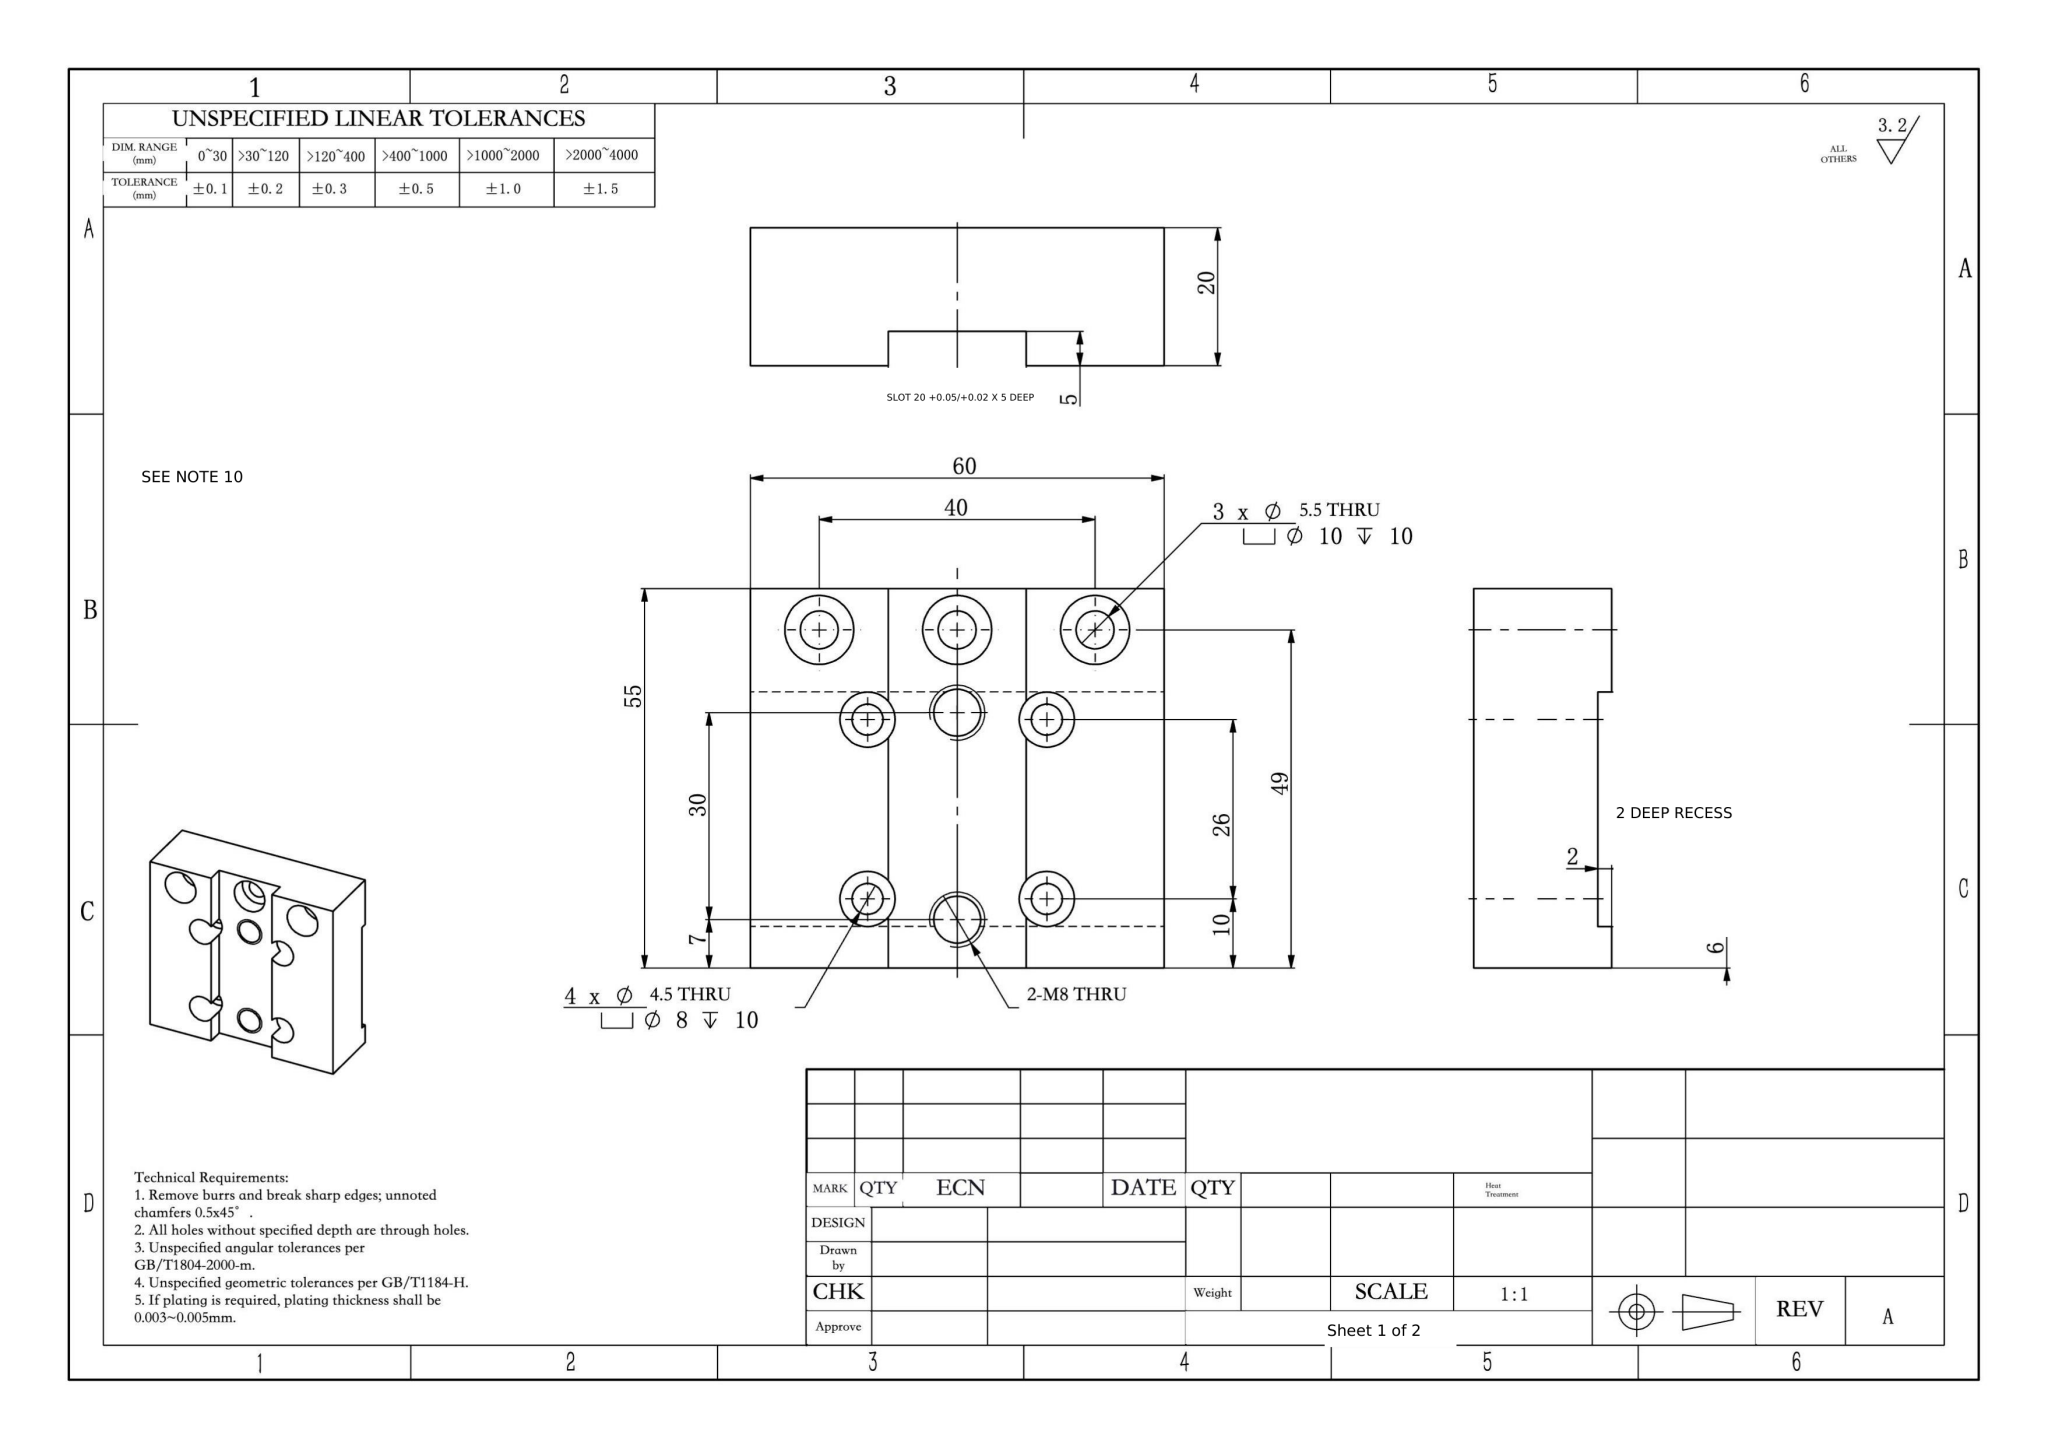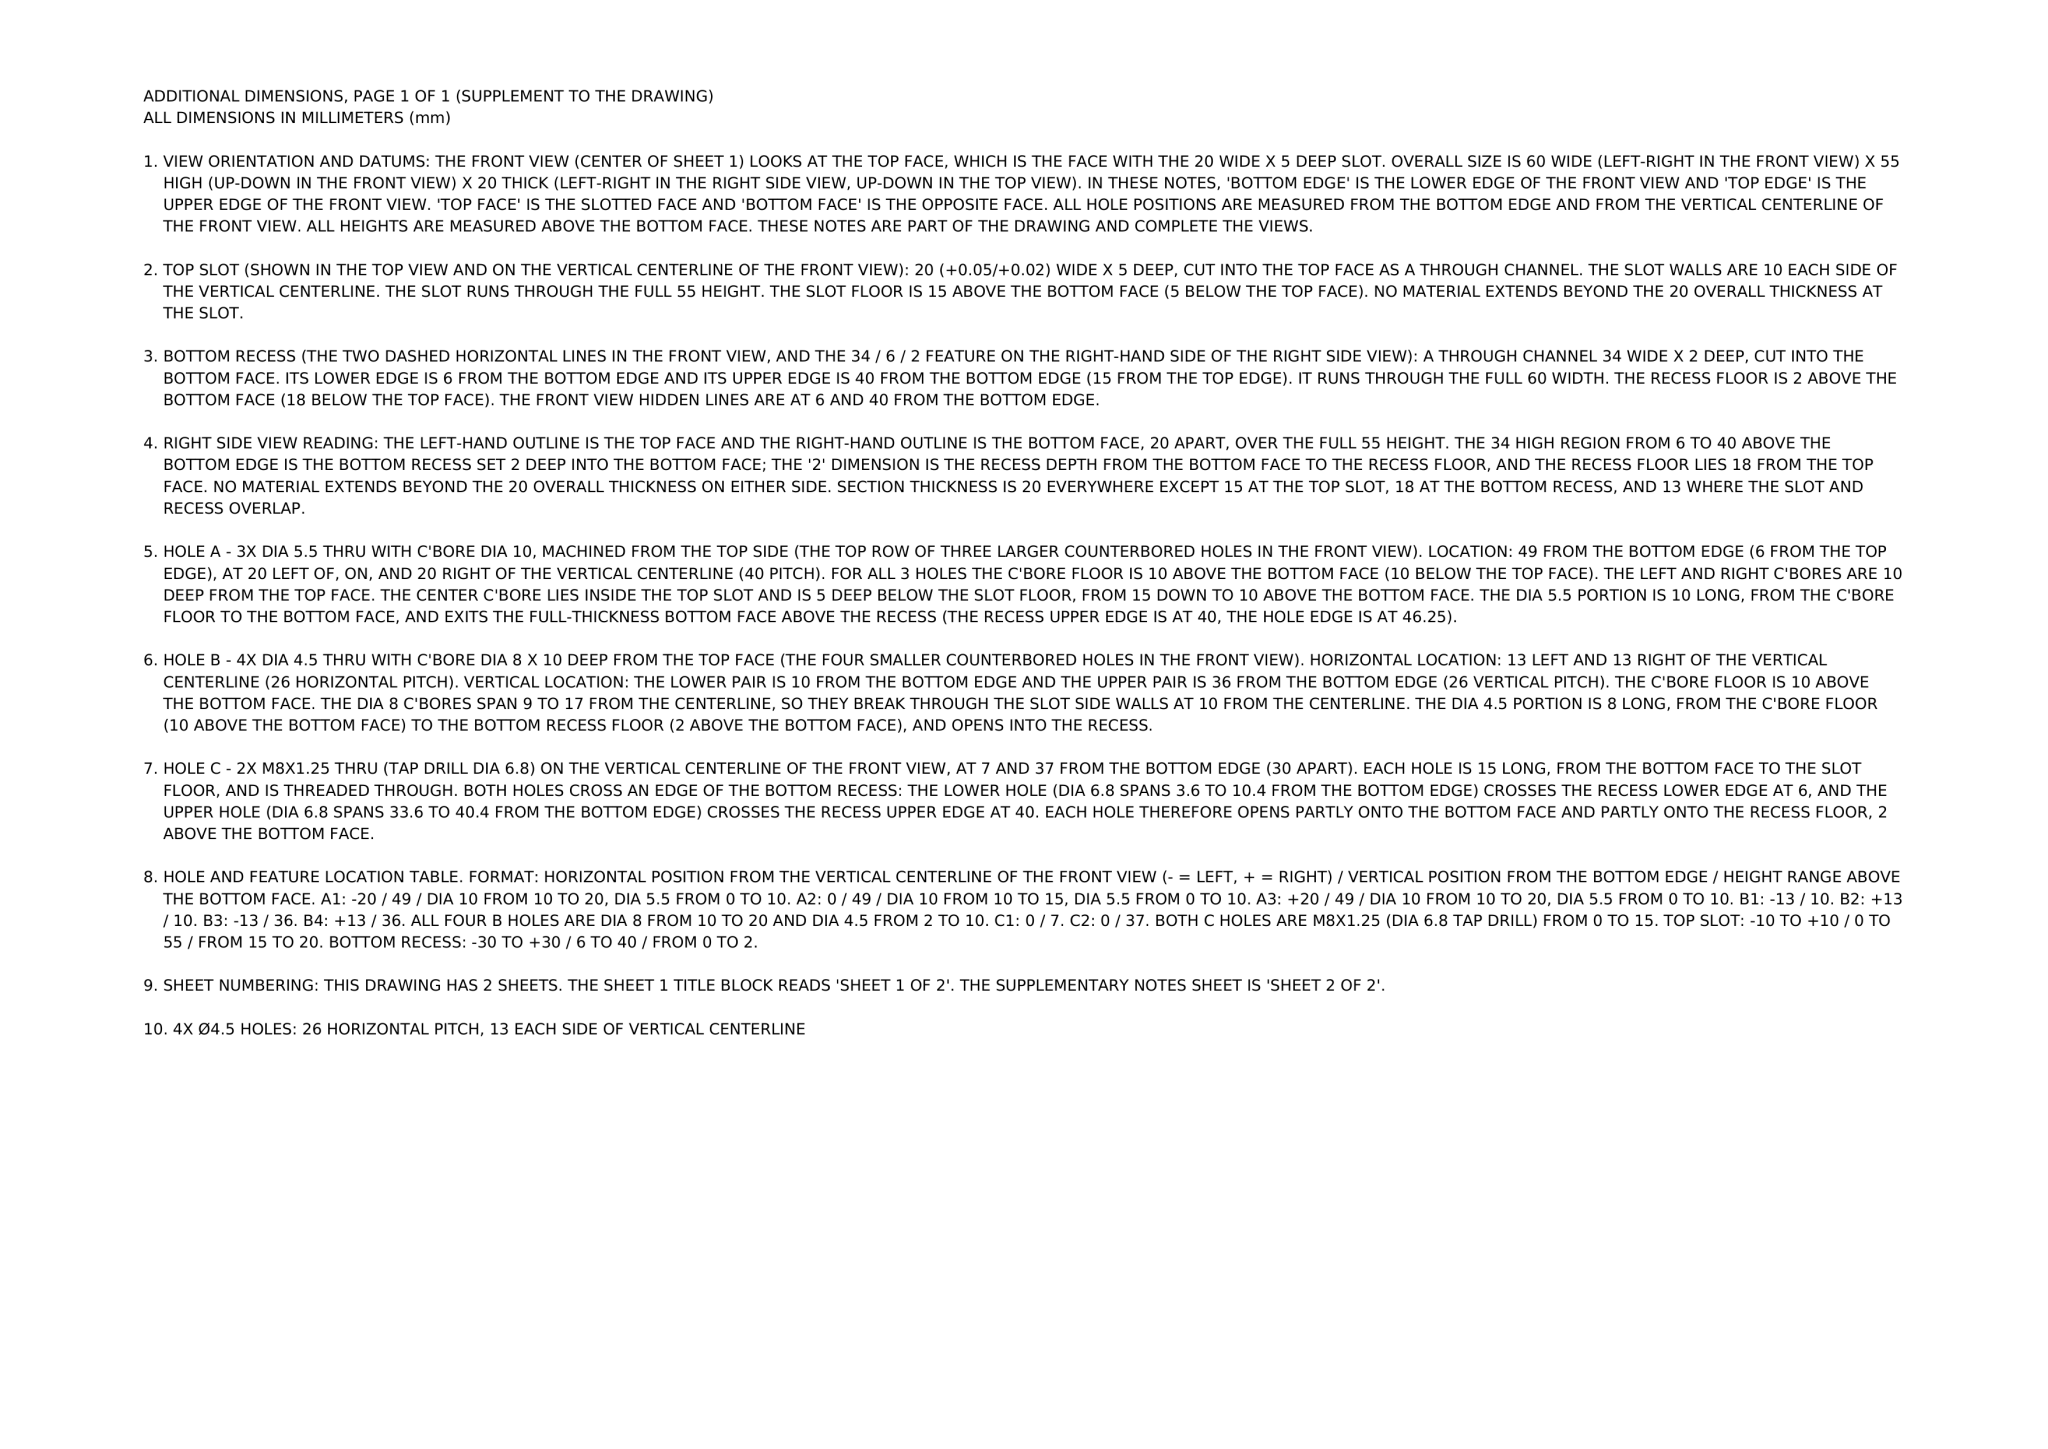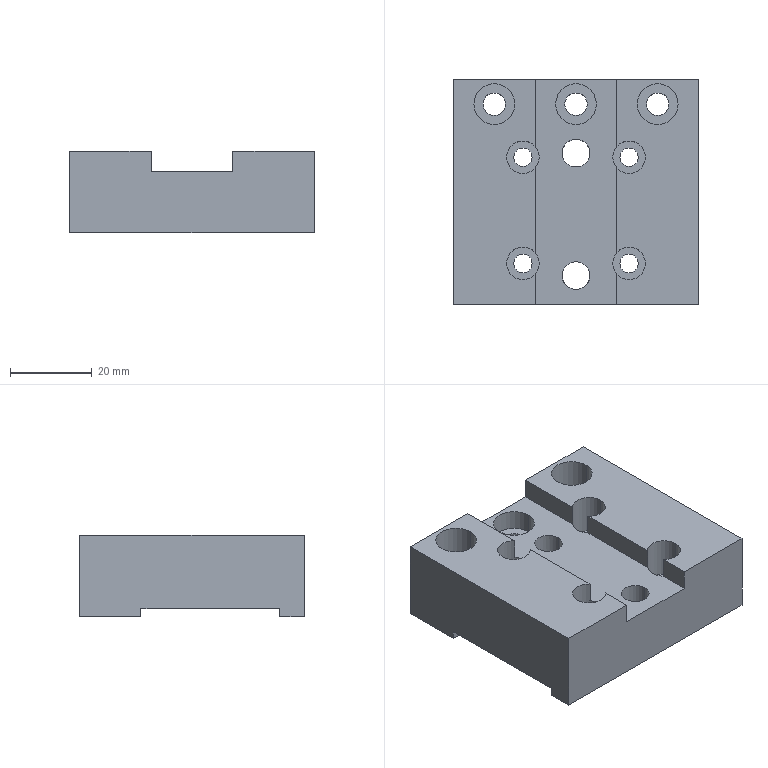Part | NX | mm | 1 solid | 59 faces | box 60 x 55 x 20 mm | volume 50328 mm3 | cylinder 32 | plane 27 | commonest cylinder face diameters 8 x8 4.5 x8 10 x6 5.5 x6 6.8 x4